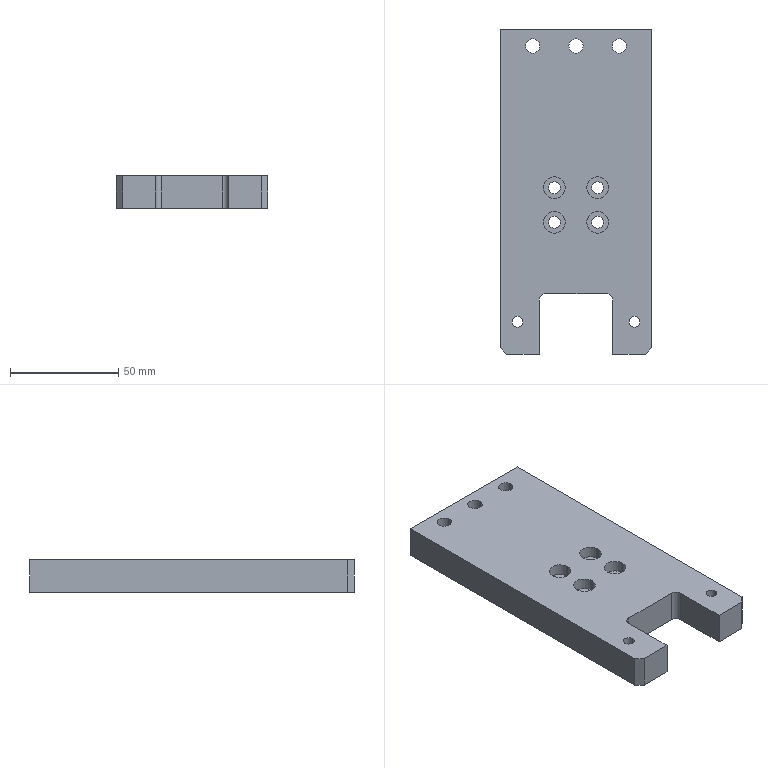Part | SolidWorks | mm | 1 solid | 53 faces | box 70 x 150 x 15 mm | volume 137238 mm3 | cylinder 34 | plane 19 | commonest cylinder face diameters 10 x8 5.5 x8 11 x6 6.6 x6 5 x4 6 x2
build123d program:
from build123d import *

# Parameters (mm, degrees)
BOSS_EXTRUDE1_DEPTH                             = 15
FILLET1_R                                       = 3
M6_TAPPED_HOLE1_D                               = 5
CHAMFER1_SIZE                                   = 3
M6_HEX_SOCKET_HEAD_CAP_SCREW_CBORE1_D           = 6.6
M6_HEX_SOCKET_HEAD_CAP_SCREW_CBORE1_CBORE_D     = 11
M6_HEX_SOCKET_HEAD_CAP_SCREW_CBORE1_CBORE_DEPTH = 6.4
M5_HEX_SOCKET_HEAD_CAP_SCREW_CBORE1_D           = 5.5
M5_HEX_SOCKET_HEAD_CAP_SCREW_CBORE1_CBORE_D     = 10
M5_HEX_SOCKET_HEAD_CAP_SCREW_CBORE1_CBORE_DEPTH = 5.4


with BuildPart() as part:
    # Sketch1 → Boss-Extrude1 (new body)
    with BuildSketch(Plane.XY):
        Polygon((-2752.108, -28.934), (-2822.108, -28.934), (-2822.108, -178.934), (-2804.108, -178.934), (-2804.108, -150.934), (-2770.108, -150.934), (-2770.108, -178.934), (-2752.108, -178.934), align=None)
    extrude(amount=BOSS_EXTRUDE1_DEPTH)

    # Fillet1
    fillet1_edges = [part.edges().sort_by_distance(p)[0] for p in [
        (-2770.108, -150.934, 7.5),
        (-2804.108, -150.934, 7.5),
    ]]
    fillet(fillet1_edges, radius=FILLET1_R)

    # M6 Tapped Hole1 (through all)
    with Locations(Plane.XY.offset(15)):
        with Locations((-2760.108, -163.934), (-2814.108, -163.934)):
            Hole(M6_TAPPED_HOLE1_D / 2)

    # Chamfer1
    chamfer1_edges = [part.edges().sort_by_distance(p)[0] for p in [
        (-2822.108, -178.934, 7.5),
        (-2752.108, -178.934, 7.5),
    ]]
    chamfer(chamfer1_edges, length=CHAMFER1_SIZE)

    # M6 Hex Socket Head Cap Screw CBORE1 (through all)
    with Locations(Plane(origin=(0, 0, 0), x_dir=(-1, 0, 0), z_dir=(0, 0, -1))):
        with Locations((2787.108, -36.434), (2767.108, -36.434), (2807.108, -36.434)):
            CounterBoreHole(M6_HEX_SOCKET_HEAD_CAP_SCREW_CBORE1_D / 2, M6_HEX_SOCKET_HEAD_CAP_SCREW_CBORE1_CBORE_D / 2, M6_HEX_SOCKET_HEAD_CAP_SCREW_CBORE1_CBORE_DEPTH)

    # M5 Hex Socket Head Cap Screw CBORE1 (through all)
    with Locations(Plane.XY.offset(15)):
        with Locations((-2777.108, -117.934), (-2797.108, -117.934), (-2797.108, -101.934), (-2777.108, -101.934)):
            CounterBoreHole(M5_HEX_SOCKET_HEAD_CAP_SCREW_CBORE1_D / 2, M5_HEX_SOCKET_HEAD_CAP_SCREW_CBORE1_CBORE_D / 2, M5_HEX_SOCKET_HEAD_CAP_SCREW_CBORE1_CBORE_DEPTH)


solid = part.part